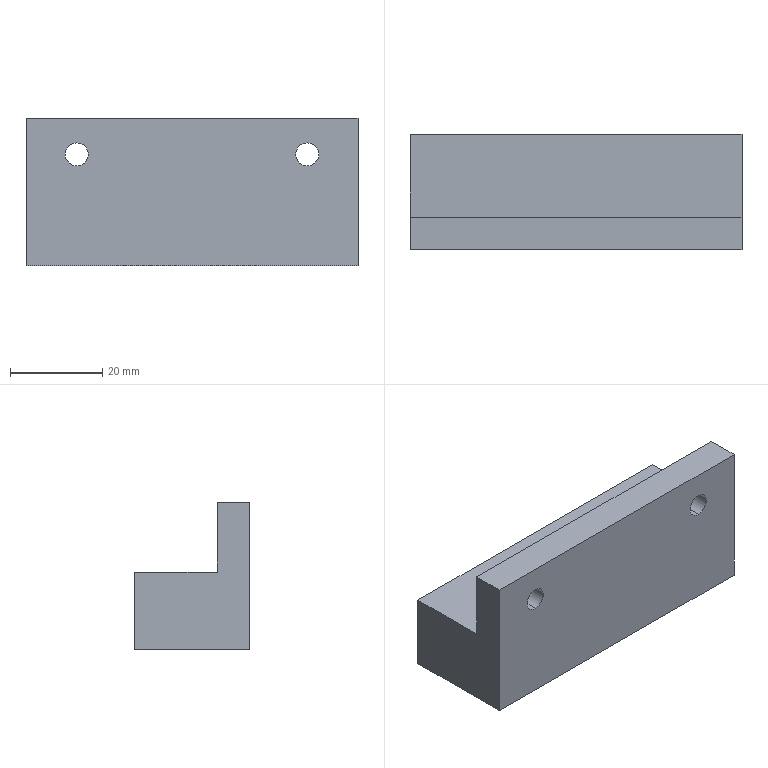Component | SolidWorks | LegSupport2-1 | 1 solid | 20 faces | box 72 x 25 x 32 mm | volume 37108 mm3 | cylinder 8 | plane 8 | cone 4 | commonest cylinder face diameters 5 x8
build123d program:
from build123d import *

# Parameters (mm, degrees)
SKETCH1_W             = 72
SKETCH1_H             = 32
BOSS_EXTRUDE1_DEPTH   = 25
SKETCH2_W             = 72
SKETCH2_H             = 15.16
CUT_EXTRUDE1_DEPTH    = 18
M5_TAPPED_HOLE1_D     = 5
M5_TAPPED_HOLE1_DEPTH = 14
M5_TAPPED_HOLE1_TIP   = 1.502
SKETCH7_R             = 2.5
CUT_EXTRUDE2_DEPTH    = 44.313


with BuildPart() as part:
    # Sketch1 → Boss-Extrude1 (new body)
    with BuildSketch(Plane(origin=(0, 0, 0), x_dir=(1, 0, 0), z_dir=(0, 1, 0))):
        Rectangle(SKETCH1_W, SKETCH1_H)
    extrude(amount=BOSS_EXTRUDE1_DEPTH)

    # Sketch2 → Cut-Extrude1 (cut)
    with BuildSketch(Plane(origin=(0, 25, 0), x_dir=(1, 0, 0), z_dir=(0, 1, 0))):
        with Locations((0, 8.42)):
            Rectangle(SKETCH2_W, SKETCH2_H)
    extrude(amount=-CUT_EXTRUDE1_DEPTH, mode=Mode.SUBTRACT)

    # M5 Tapped Hole1
    with Locations(Plane(origin=(-25, 25, 8.16), x_dir=(0, 0, 1), z_dir=(0, 1, 0))):
        with Locations((0, 0), (0, 50)):
            Hole(M5_TAPPED_HOLE1_D / 2, depth=M5_TAPPED_HOLE1_DEPTH)
            with Locations((0, 0, -(M5_TAPPED_HOLE1_DEPTH + M5_TAPPED_HOLE1_TIP / 2))):  # 118° drill point
                Cone(0, M5_TAPPED_HOLE1_D / 2, M5_TAPPED_HOLE1_TIP, mode=Mode.SUBTRACT)

    # Sketch7 → Cut-Extrude2 (cut, through all)
    with BuildSketch(Plane(origin=(0, 7, 0), x_dir=(1, 0, 0), z_dir=(0, 1, 0))):
        with Locations(Location((-25, 8.16, 0), (0, 0, 270))):
            Circle(SKETCH7_R)
        with Locations(Location((25, 8.16, 0), (0, 0, 90))):
            Circle(SKETCH7_R)
    extrude(amount=-CUT_EXTRUDE2_DEPTH, mode=Mode.SUBTRACT)


solid = part.part

# Placed as in the assembly
solid = solid.moved(Location((-96.534, 53.266, -102.347), (-180, 0, 180)))
STEP:
#1=COLOUR_RGB('',0.7922,0.8196,0.9333);
#2=FILL_AREA_STYLE_COLOUR('',#1);
#3=FILL_AREA_STYLE('',(#2));
#4=SURFACE_STYLE_FILL_AREA(#3);
#5=SURFACE_SIDE_STYLE('',(#4));
#6=SURFACE_STYLE_USAGE(.BOTH.,#5);
#7=PRESENTATION_STYLE_ASSIGNMENT((#6));
#8=CARTESIAN_POINT('',(-4.785,2.097,-3.61));
#9=VERTEX_POINT('',#8);
#10=CARTESIAN_POINT('',(-4.785,2.097,-3.807));
#11=VERTEX_POINT('',#10);
#12=CARTESIAN_POINT('',(-4.785,2.097,-3.708));
#13=DIRECTION('',(0.,1.,0.));
#14=DIRECTION('',(0.,0.,1.));
#15=AXIS2_PLACEMENT_3D('',#12,#13,#14);
#16=CIRCLE('',#15,0.09843);
#17=EDGE_CURVE('',#9,#11,#16,.T.);
#18=ORIENTED_EDGE('',*,*,#17,.F.);
#19=CARTESIAN_POINT('',(-4.785,2.373,-3.61));
#20=VERTEX_POINT('',#19);
#21=CARTESIAN_POINT('',(-4.785,2.097,-3.61));
#22=DIRECTION('',(0.,1.,0.));
#23=VECTOR('',#22,39.37);
#24=LINE('',#21,#23);
#25=EDGE_CURVE('',#9,#20,#24,.T.);
#26=ORIENTED_EDGE('',*,*,#25,.T.);
#27=CARTESIAN_POINT('',(-4.785,2.373,-3.807));
#28=VERTEX_POINT('',#27);
#29=CARTESIAN_POINT('',(-4.785,2.373,-3.708));
#30=DIRECTION('',(0.,1.,0.));
#31=DIRECTION('',(0.,0.,1.));
#32=AXIS2_PLACEMENT_3D('',#29,#30,#31);
#33=CIRCLE('',#32,0.09843);
#34=EDGE_CURVE('',#20,#28,#33,.T.);
#35=ORIENTED_EDGE('',*,*,#34,.T.);
#36=CARTESIAN_POINT('',(-4.785,2.097,-3.807));
#37=DIRECTION('',(0.,1.,0.));
#38=VECTOR('',#37,39.37);
#39=LINE('',#36,#38);
#40=EDGE_CURVE('',#11,#28,#39,.T.);
#41=ORIENTED_EDGE('',*,*,#40,.F.);
#42=EDGE_LOOP('',(#18,#26,#35,#41));
#43=FACE_OUTER_BOUND('',#42,.T.);
#44=CARTESIAN_POINT('',(-4.785,2.097,-3.708));
#45=DIRECTION('',(0.,1.,0.));
#46=DIRECTION('',(0.,0.,-1.));
#47=AXIS2_PLACEMENT_3D('',#44,#45,#46);
#48=CYLINDRICAL_SURFACE('',#47,0.09843);
#49=ADVANCED_FACE('',(#43),#48,.F.);
#50=CARTESIAN_POINT('',(-2.816,2.097,-3.61));
#51=VERTEX_POINT('',#50);
#52=CARTESIAN_POINT('',(-2.816,2.097,-3.807));
#53=VERTEX_POINT('',#52);
#54=CARTESIAN_POINT('',(-2.816,2.097,-3.708));
#55=DIRECTION('',(0.,1.,0.));
#56=DIRECTION('',(0.,0.,-1.));
#57=AXIS2_PLACEMENT_3D('',#54,#55,#56);
#58=CIRCLE('',#57,0.09843);
#59=EDGE_CURVE('',#51,#53,#58,.T.);
#60=ORIENTED_EDGE('',*,*,#59,.F.);
#61=CARTESIAN_POINT('',(-2.816,2.373,-3.61));
#62=VERTEX_POINT('',#61);
#63=CARTESIAN_POINT('',(-2.816,2.097,-3.61));
#64=DIRECTION('',(0.,1.,0.));
#65=VECTOR('',#64,39.37);
#66=LINE('',#63,#65);
#67=EDGE_CURVE('',#51,#62,#66,.T.);
#68=ORIENTED_EDGE('',*,*,#67,.T.);
#69=CARTESIAN_POINT('',(-2.816,2.373,-3.807));
#70=VERTEX_POINT('',#69);
#71=CARTESIAN_POINT('',(-2.816,2.373,-3.708));
#72=DIRECTION('',(0.,1.,0.));
#73=DIRECTION('',(0.,0.,-1.));
#74=AXIS2_PLACEMENT_3D('',#71,#72,#73);
#75=CIRCLE('',#74,0.09843);
#76=EDGE_CURVE('',#62,#70,#75,.T.);
#77=ORIENTED_EDGE('',*,*,#76,.T.);
#78=CARTESIAN_POINT('',(-2.816,2.097,-3.807));
#79=DIRECTION('',(0.,1.,0.));
#80=VECTOR('',#79,39.37);
#81=LINE('',#78,#80);
#82=EDGE_CURVE('',#53,#70,#81,.T.);
#83=ORIENTED_EDGE('',*,*,#82,.F.);
#84=EDGE_LOOP('',(#60,#68,#77,#83));
#85=FACE_OUTER_BOUND('',#84,.T.);
#86=CARTESIAN_POINT('',(-2.816,2.097,-3.708));
#87=DIRECTION('',(0.,1.,0.));
#88=DIRECTION('',(0.,0.,-1.));
#89=AXIS2_PLACEMENT_3D('',#86,#87,#88);
#90=CYLINDRICAL_SURFACE('',#89,0.09843);
#91=ADVANCED_FACE('',(#85),#90,.F.);
#92=CARTESIAN_POINT('',(-2.816,2.53,-4.252));
#93=VERTEX_POINT('',#92);
#94=CARTESIAN_POINT('',(-2.816,2.53,-4.449));
#95=VERTEX_POINT('',#94);
#96=CARTESIAN_POINT('',(-2.816,2.53,-4.351));
#97=DIRECTION('',(0.,1.,0.));
#98=DIRECTION('',(0.,0.,-1.));
#99=AXIS2_PLACEMENT_3D('',#96,#97,#98);
#100=CIRCLE('',#99,0.09843);
#101=EDGE_CURVE('',#93,#95,#100,.T.);
#102=ORIENTED_EDGE('',*,*,#101,.F.);
#103=CARTESIAN_POINT('',(-2.816,3.081,-4.252));
#104=VERTEX_POINT('',#103);
#105=CARTESIAN_POINT('',(-2.816,3.081,-4.252));
#106=DIRECTION('',(0.,1.,0.));
#107=VECTOR('',#106,39.37);
#108=LINE('',#105,#107);
#109=EDGE_CURVE('',#93,#104,#108,.T.);
#110=ORIENTED_EDGE('',*,*,#109,.T.);
#111=CARTESIAN_POINT('',(-2.816,3.081,-4.449));
#112=VERTEX_POINT('',#111);
#113=CARTESIAN_POINT('',(-2.816,3.081,-4.351));
#114=DIRECTION('',(0.,1.,0.));
#115=DIRECTION('',(0.,0.,-1.));
#116=AXIS2_PLACEMENT_3D('',#113,#114,#115);
#117=CIRCLE('',#116,0.09843);
#118=EDGE_CURVE('',#104,#112,#117,.T.);
#119=ORIENTED_EDGE('',*,*,#118,.T.);
#120=CARTESIAN_POINT('',(-2.816,3.081,-4.449));
#121=DIRECTION('',(0.,1.,0.));
#122=VECTOR('',#121,39.37);
#123=LINE('',#120,#122);
#124=EDGE_CURVE('',#95,#112,#123,.T.);
#125=ORIENTED_EDGE('',*,*,#124,.F.);
#126=EDGE_LOOP('',(#102,#110,#119,#125));
#127=FACE_OUTER_BOUND('',#126,.T.);
#128=CARTESIAN_POINT('',(-2.816,3.081,-4.351));
#129=DIRECTION('',(0.,1.,0.));
#130=DIRECTION('',(0.,0.,-1.));
#131=AXIS2_PLACEMENT_3D('',#128,#129,#130);
#132=CYLINDRICAL_SURFACE('',#131,0.09843);
#133=ADVANCED_FACE('',(#127),#132,.F.);
#134=CARTESIAN_POINT('',(-2.816,2.471,-4.351));
#135=VERTEX_POINT('',#134);
#136=CARTESIAN_POINT('',(-2.816,2.53,-4.449));
#137=DIRECTION('',(-0.,0.515,-0.8572));
#138=VECTOR('',#137,39.37);
#139=LINE('',#136,#138);
#140=EDGE_CURVE('',#135,#95,#139,.T.);
#141=ORIENTED_EDGE('',*,*,#140,.F.);
#142=CARTESIAN_POINT('',(-2.816,2.53,-4.252));
#143=DIRECTION('',(0.,0.515,0.8572));
#144=VECTOR('',#143,39.37);
#145=LINE('',#142,#144);
#146=EDGE_CURVE('',#135,#93,#145,.T.);
#147=ORIENTED_EDGE('',*,*,#146,.T.);
#148=ORIENTED_EDGE('',*,*,#101,.T.);
#149=EDGE_LOOP('',(#141,#147,#148));
#150=FACE_OUTER_BOUND('',#149,.T.);
#151=CARTESIAN_POINT('',(-2.816,2.53,-4.351));
#152=DIRECTION('',(0.,1.,0.));
#153=DIRECTION('',(0.,0.,-1.));
#154=AXIS2_PLACEMENT_3D('',#151,#152,#153);
#155=CONICAL_SURFACE('',#154,0.09843,1.03);
#156=ADVANCED_FACE('',(#150),#155,.F.);
#157=CARTESIAN_POINT('',(-4.785,2.53,-4.252));
#158=VERTEX_POINT('',#157);
#159=CARTESIAN_POINT('',(-4.785,2.53,-4.449));
#160=VERTEX_POINT('',#159);
#161=CARTESIAN_POINT('',(-4.785,2.53,-4.351));
#162=DIRECTION('',(0.,1.,0.));
#163=DIRECTION('',(0.,0.,-1.));
#164=AXIS2_PLACEMENT_3D('',#161,#162,#163);
#165=CIRCLE('',#164,0.09843);
#166=EDGE_CURVE('',#158,#160,#165,.T.);
#167=ORIENTED_EDGE('',*,*,#166,.F.);
#168=CARTESIAN_POINT('',(-4.785,3.081,-4.252));
#169=VERTEX_POINT('',#168);
#170=CARTESIAN_POINT('',(-4.785,3.081,-4.252));
#171=DIRECTION('',(0.,1.,0.));
#172=VECTOR('',#171,39.37);
#173=LINE('',#170,#172);
#174=EDGE_CURVE('',#158,#169,#173,.T.);
#175=ORIENTED_EDGE('',*,*,#174,.T.);
#176=CARTESIAN_POINT('',(-4.785,3.081,-4.449));
#177=VERTEX_POINT('',#176);
#178=CARTESIAN_POINT('',(-4.785,3.081,-4.351));
#179=DIRECTION('',(0.,1.,0.));
#180=DIRECTION('',(0.,0.,-1.));
#181=AXIS2_PLACEMENT_3D('',#178,#179,#180);
#182=CIRCLE('',#181,0.09843);
#183=EDGE_CURVE('',#169,#177,#182,.T.);
#184=ORIENTED_EDGE('',*,*,#183,.T.);
#185=CARTESIAN_POINT('',(-4.785,3.081,-4.449));
#186=DIRECTION('',(0.,1.,0.));
#187=VECTOR('',#186,39.37);
#188=LINE('',#185,#187);
#189=EDGE_CURVE('',#160,#177,#188,.T.);
#190=ORIENTED_EDGE('',*,*,#189,.F.);
#191=EDGE_LOOP('',(#167,#175,#184,#190));
#192=FACE_OUTER_BOUND('',#191,.T.);
#193=CARTESIAN_POINT('',(-4.785,3.081,-4.351));
#194=DIRECTION('',(0.,1.,0.));
#195=DIRECTION('',(0.,0.,-1.));
#196=AXIS2_PLACEMENT_3D('',#193,#194,#195);
#197=CYLINDRICAL_SURFACE('',#196,0.09843);
#198=ADVANCED_FACE('',(#192),#197,.F.);
#199=CARTESIAN_POINT('',(-4.785,2.471,-4.351));
#200=VERTEX_POINT('',#199);
#201=CARTESIAN_POINT('',(-4.785,2.53,-4.449));
#202=DIRECTION('',(-0.,0.515,-0.8572));
#203=VECTOR('',#202,39.37);
#204=LINE('',#201,#203);
#205=EDGE_CURVE('',#200,#160,#204,.T.);
#206=ORIENTED_EDGE('',*,*,#205,.F.);
#207=CARTESIAN_POINT('',(-4.785,2.53,-4.252));
#208=DIRECTION('',(0.,0.515,0.8572));
#209=VECTOR('',#208,39.37);
#210=LINE('',#207,#209);
#211=EDGE_CURVE('',#200,#158,#210,.T.);
#212=ORIENTED_EDGE('',*,*,#211,.T.);
#213=ORIENTED_EDGE('',*,*,#166,.T.);
#214=EDGE_LOOP('',(#206,#212,#213));
#215=FACE_OUTER_BOUND('',#214,.T.);
#216=CARTESIAN_POINT('',(-4.785,2.53,-4.351));
#217=DIRECTION('',(0.,1.,0.));
#218=DIRECTION('',(0.,0.,-1.));
#219=AXIS2_PLACEMENT_3D('',#216,#217,#218);
#220=CONICAL_SURFACE('',#219,0.09843,1.03);
#221=ADVANCED_FACE('',(#215),#220,.F.);
#222=CARTESIAN_POINT('',(-5.218,2.373,-3.399));
#223=VERTEX_POINT('',#222);
#224=CARTESIAN_POINT('',(-2.383,2.373,-3.399));
#225=VERTEX_POINT('',#224);
#226=CARTESIAN_POINT('',(-2.383,2.373,-3.399));
#227=DIRECTION('',(1.,0.,-0.));
#228=VECTOR('',#227,39.37);
#229=LINE('',#226,#228);
#230=EDGE_CURVE('',#223,#225,#229,.T.);
#231=ORIENTED_EDGE('',*,*,#230,.F.);
#232=CARTESIAN_POINT('',(-5.218,2.097,-3.399));
#233=VERTEX_POINT('',#232);
#234=CARTESIAN_POINT('',(-5.218,3.081,-3.399));
#235=DIRECTION('',(0.,-1.,0.));
#236=VECTOR('',#235,39.37);
#237=LINE('',#234,#236);
#238=EDGE_CURVE('',#223,#233,#237,.T.);
#239=ORIENTED_EDGE('',*,*,#238,.T.);
#240=CARTESIAN_POINT('',(-2.383,2.097,-3.399));
#241=VERTEX_POINT('',#240);
#242=CARTESIAN_POINT('',(-2.383,2.097,-3.399));
#243=DIRECTION('',(1.,0.,-0.));
#244=VECTOR('',#243,39.37);
#245=LINE('',#242,#244);
#246=EDGE_CURVE('',#233,#241,#245,.T.);
#247=ORIENTED_EDGE('',*,*,#246,.T.);
#248=CARTESIAN_POINT('',(-2.383,3.081,-3.399));
#249=DIRECTION('',(0.,-1.,0.));
#250=VECTOR('',#249,39.37);
#251=LINE('',#248,#250);
#252=EDGE_CURVE('',#225,#241,#251,.T.);
#253=ORIENTED_EDGE('',*,*,#252,.F.);
#254=EDGE_LOOP('',(#231,#239,#247,#253));
#255=FACE_OUTER_BOUND('',#254,.T.);
#256=CARTESIAN_POINT('',(-2.383,3.081,-3.399));
#257=DIRECTION('',(-0.,0.,-1.));
#258=DIRECTION('',(-1.,0.,0.));
#259=AXIS2_PLACEMENT_3D('',#256,#257,#258);
#260=PLANE('',#259);
#261=ADVANCED_FACE('',(#255),#260,.F.);
#262=CARTESIAN_POINT('',(-5.218,2.373,-3.996));
#263=VERTEX_POINT('',#262);
#264=CARTESIAN_POINT('',(-5.218,2.373,-3.399));
#265=DIRECTION('',(0.,0.,1.));
#266=VECTOR('',#265,39.37);
#267=LINE('',#264,#266);
#268=EDGE_CURVE('',#263,#223,#267,.T.);
#269=ORIENTED_EDGE('',*,*,#268,.F.);
#270=CARTESIAN_POINT('',(-5.218,3.081,-3.996));
#271=VERTEX_POINT('',#270);
#272=CARTESIAN_POINT('',(-5.218,2.373,-3.996));
#273=DIRECTION('',(0.,1.,0.));
#274=VECTOR('',#273,39.37);
#275=LINE('',#272,#274);
#276=EDGE_CURVE('',#263,#271,#275,.T.);
#277=ORIENTED_EDGE('',*,*,#276,.T.);
#278=CARTESIAN_POINT('',(-5.218,3.081,-4.659));
#279=VERTEX_POINT('',#278);
#280=CARTESIAN_POINT('',(-5.218,3.081,-3.399));
#281=DIRECTION('',(0.,0.,1.));
#282=VECTOR('',#281,39.37);
#283=LINE('',#280,#282);
#284=EDGE_CURVE('',#279,#271,#283,.T.);
#285=ORIENTED_EDGE('',*,*,#284,.F.);
#286=CARTESIAN_POINT('',(-5.218,2.097,-4.659));
#287=VERTEX_POINT('',#286);
#288=CARTESIAN_POINT('',(-5.218,3.081,-4.659));
#289=DIRECTION('',(0.,-1.,0.));
#290=VECTOR('',#289,39.37);
#291=LINE('',#288,#290);
#292=EDGE_CURVE('',#279,#287,#291,.T.);
#293=ORIENTED_EDGE('',*,*,#292,.T.);
#294=CARTESIAN_POINT('',(-5.218,2.097,-3.399));
#295=DIRECTION('',(0.,0.,1.));
#296=VECTOR('',#295,39.37);
#297=LINE('',#294,#296);
#298=EDGE_CURVE('',#287,#233,#297,.T.);
#299=ORIENTED_EDGE('',*,*,#298,.T.);
#300=ORIENTED_EDGE('',*,*,#238,.F.);
#301=EDGE_LOOP('',(#269,#277,#285,#293,#299,#300));
#302=FACE_OUTER_BOUND('',#301,.T.);
#303=CARTESIAN_POINT('',(-5.218,3.081,-3.399));
#304=DIRECTION('',(1.,0.,-0.));
#305=DIRECTION('',(-0.,0.,-1.));
#306=AXIS2_PLACEMENT_3D('',#303,#304,#305);
#307=PLANE('',#306);
#308=ADVANCED_FACE('',(#302),#307,.F.);
#309=CARTESIAN_POINT('',(-2.383,3.081,-3.996));
#310=VERTEX_POINT('',#309);
#311=CARTESIAN_POINT('',(-2.383,3.081,-4.659));
#312=VERTEX_POINT('',#311);
#313=CARTESIAN_POINT('',(-2.383,3.081,-3.399));
#314=DIRECTION('',(-0.,0.,-1.));
#315=VECTOR('',#314,39.37);
#316=LINE('',#313,#315);
#317=EDGE_CURVE('',#310,#312,#316,.T.);
#318=ORIENTED_EDGE('',*,*,#317,.F.);
#319=CARTESIAN_POINT('',(-2.383,2.373,-3.996));
#320=VERTEX_POINT('',#319);
#321=CARTESIAN_POINT('',(-2.383,2.373,-3.996));
#322=DIRECTION('',(0.,1.,0.));
#323=VECTOR('',#322,39.37);
#324=LINE('',#321,#323);
#325=EDGE_CURVE('',#320,#310,#324,.T.);
#326=ORIENTED_EDGE('',*,*,#325,.F.);
#327=CARTESIAN_POINT('',(-2.383,2.373,-3.399));
#328=DIRECTION('',(-0.,0.,-1.));
#329=VECTOR('',#328,39.37);
#330=LINE('',#327,#329);
#331=EDGE_CURVE('',#225,#320,#330,.T.);
#332=ORIENTED_EDGE('',*,*,#331,.F.);
#333=ORIENTED_EDGE('',*,*,#252,.T.);
#334=CARTESIAN_POINT('',(-2.383,2.097,-4.659));
#335=VERTEX_POINT('',#334);
#336=CARTESIAN_POINT('',(-2.383,2.097,-3.399));
#337=DIRECTION('',(-0.,0.,-1.));
#338=VECTOR('',#337,39.37);
#339=LINE('',#336,#338);
#340=EDGE_CURVE('',#241,#335,#339,.T.);
#341=ORIENTED_EDGE('',*,*,#340,.T.);
#342=CARTESIAN_POINT('',(-2.383,3.081,-4.659));
#343=DIRECTION('',(0.,-1.,0.));
#344=VECTOR('',#343,39.37);
#345=LINE('',#342,#344);
#346=EDGE_CURVE('',#312,#335,#345,.T.);
#347=ORIENTED_EDGE('',*,*,#346,.F.);
#348=EDGE_LOOP('',(#318,#326,#332,#333,#341,#347));
#349=FACE_OUTER_BOUND('',#348,.T.);
#350=CARTESIAN_POINT('',(-2.383,3.081,-3.399));
#351=DIRECTION('',(-1.,0.,0.));
#352=DIRECTION('',(0.,0.,1.));
#353=AXIS2_PLACEMENT_3D('',#350,#351,#352);
#354=PLANE('',#353);
#355=ADVANCED_FACE('',(#349),#354,.F.);
#356=CARTESIAN_POINT('',(-2.383,2.097,-4.659));
#357=DIRECTION('',(-1.,0.,0.));
#358=VECTOR('',#357,39.37);
#359=LINE('',#356,#358);
#360=EDGE_CURVE('',#335,#287,#359,.T.);
#361=ORIENTED_EDGE('',*,*,#360,.T.);
#362=ORIENTED_EDGE('',*,*,#292,.F.);
#363=CARTESIAN_POINT('',(-2.383,3.081,-4.659));
#364=DIRECTION('',(-1.,0.,0.));
#365=VECTOR('',#364,39.37);
#366=LINE('',#363,#365);
#367=EDGE_CURVE('',#312,#279,#366,.T.);
#368=ORIENTED_EDGE('',*,*,#367,.F.);
#369=ORIENTED_EDGE('',*,*,#346,.T.);
#370=EDGE_LOOP('',(#361,#362,#368,#369));
#371=FACE_OUTER_BOUND('',#370,.T.);
#372=CARTESIAN_POINT('',(-2.383,3.081,-4.659));
#373=DIRECTION('',(0.,0.,1.));
#374=DIRECTION('',(1.,0.,-0.));
#375=AXIS2_PLACEMENT_3D('',#372,#373,#374);
#376=PLANE('',#375);
#377=ADVANCED_FACE('',(#371),#376,.F.);
#378=CARTESIAN_POINT('',(-2.816,3.081,-4.351));
#379=DIRECTION('',(0.,1.,0.));
#380=DIRECTION('',(0.,0.,-1.));
#381=AXIS2_PLACEMENT_3D('',#378,#379,#380);
#382=CIRCLE('',#381,0.09843);
#383=EDGE_CURVE('',#112,#104,#382,.T.);
#384=ORIENTED_EDGE('',*,*,#383,.F.);
#385=ORIENTED_EDGE('',*,*,#118,.F.);
#386=EDGE_LOOP('',(#384,#385));
#387=FACE_BOUND('',#386,.T.);
#388=CARTESIAN_POINT('',(-4.785,3.081,-4.351));
#389=DIRECTION('',(0.,1.,0.));
#390=DIRECTION('',(0.,0.,-1.));
#391=AXIS2_PLACEMENT_3D('',#388,#389,#390);
#392=CIRCLE('',#391,0.09843);
#393=EDGE_CURVE('',#177,#169,#392,.T.);
#394=ORIENTED_EDGE('',*,*,#393,.F.);
#395=ORIENTED_EDGE('',*,*,#183,.F.);
#396=EDGE_LOOP('',(#394,#395));
#397=FACE_BOUND('',#396,.T.);
#398=CARTESIAN_POINT('',(-2.383,3.081,-3.996));
#399=DIRECTION('',(-1.,0.,0.));
#400=VECTOR('',#399,39.37);
#401=LINE('',#398,#400);
#402=EDGE_CURVE('',#310,#271,#401,.T.);
#403=ORIENTED_EDGE('',*,*,#402,.F.);
#404=ORIENTED_EDGE('',*,*,#317,.T.);
#405=ORIENTED_EDGE('',*,*,#367,.T.);
#406=ORIENTED_EDGE('',*,*,#284,.T.);
#407=EDGE_LOOP('',(#403,#404,#405,#406));
#408=FACE_OUTER_BOUND('',#407,.T.);
#409=CARTESIAN_POINT('',(-3.801,3.081,-4.029));
#410=DIRECTION('',(0.,1.,0.));
#411=DIRECTION('',(-0.,0.,-1.));
#412=AXIS2_PLACEMENT_3D('',#409,#410,#411);
#413=PLANE('',#412);
#414=ADVANCED_FACE('',(#387,#397,#408),#413,.T.);
#415=CARTESIAN_POINT('',(-4.785,2.097,-3.708));
#416=DIRECTION('',(0.,1.,0.));
#417=DIRECTION('',(0.,0.,1.));
#418=AXIS2_PLACEMENT_3D('',#415,#416,#417);
#419=CIRCLE('',#418,0.09843);
#420=EDGE_CURVE('',#11,#9,#419,.T.);
#421=ORIENTED_EDGE('',*,*,#420,.T.);
#422=ORIENTED_EDGE('',*,*,#17,.T.);
#423=EDGE_LOOP('',(#421,#422));
#424=FACE_BOUND('',#423,.T.);
#425=CARTESIAN_POINT('',(-2.816,2.097,-3.708));
#426=DIRECTION('',(0.,1.,0.));
#427=DIRECTION('',(0.,0.,-1.));
#428=AXIS2_PLACEMENT_3D('',#425,#426,#427);
#429=CIRCLE('',#428,0.09843);
#430=EDGE_CURVE('',#53,#51,#429,.T.);
#431=ORIENTED_EDGE('',*,*,#430,.T.);
#432=ORIENTED_EDGE('',*,*,#59,.T.);
#433=EDGE_LOOP('',(#431,#432));
#434=FACE_BOUND('',#433,.T.);
#435=ORIENTED_EDGE('',*,*,#298,.F.);
#436=ORIENTED_EDGE('',*,*,#360,.F.);
#437=ORIENTED_EDGE('',*,*,#340,.F.);
#438=ORIENTED_EDGE('',*,*,#246,.F.);
#439=EDGE_LOOP('',(#435,#436,#437,#438));
#440=FACE_OUTER_BOUND('',#439,.T.);
#441=CARTESIAN_POINT('',(-3.801,2.097,-4.029));
#442=DIRECTION('',(0.,1.,0.));
#443=DIRECTION('',(-0.,0.,-1.));
#444=AXIS2_PLACEMENT_3D('',#441,#442,#443);
#445=PLANE('',#444);
#446=ADVANCED_FACE('',(#424,#434,#440),#445,.F.);
#447=ORIENTED_EDGE('',*,*,#402,.T.);
#448=ORIENTED_EDGE('',*,*,#276,.F.);
#449=CARTESIAN_POINT('',(-2.383,2.373,-3.996));
#450=DIRECTION('',(-1.,0.,0.));
#451=VECTOR('',#450,39.37);
#452=LINE('',#449,#451);
#453=EDGE_CURVE('',#320,#263,#452,.T.);
#454=ORIENTED_EDGE('',*,*,#453,.F.);
#455=ORIENTED_EDGE('',*,*,#325,.T.);
#456=EDGE_LOOP('',(#447,#448,#454,#455));
#457=FACE_OUTER_BOUND('',#456,.T.);
#458=CARTESIAN_POINT('',(-2.383,2.373,-3.996));
#459=DIRECTION('',(-0.,0.,-1.));
#460=DIRECTION('',(-1.,0.,0.));
#461=AXIS2_PLACEMENT_3D('',#458,#459,#460);
#462=PLANE('',#461);
#463=ADVANCED_FACE('',(#457),#462,.F.);
#464=CARTESIAN_POINT('',(-4.785,2.373,-3.708));
#465=DIRECTION('',(0.,1.,0.));
#466=DIRECTION('',(0.,0.,1.));
#467=AXIS2_PLACEMENT_3D('',#464,#465,#466);
#468=CIRCLE('',#467,0.09843);
#469=EDGE_CURVE('',#28,#20,#468,.T.);
#470=ORIENTED_EDGE('',*,*,#469,.F.);
#471=ORIENTED_EDGE('',*,*,#34,.F.);
#472=EDGE_LOOP('',(#470,#471));
#473=FACE_BOUND('',#472,.T.);
#474=CARTESIAN_POINT('',(-2.816,2.373,-3.708));
#475=DIRECTION('',(0.,1.,0.));
#476=DIRECTION('',(0.,0.,-1.));
#477=AXIS2_PLACEMENT_3D('',#474,#475,#476);
#478=CIRCLE('',#477,0.09843);
#479=EDGE_CURVE('',#70,#62,#478,.T.);
#480=ORIENTED_EDGE('',*,*,#479,.F.);
#481=ORIENTED_EDGE('',*,*,#76,.F.);
#482=EDGE_LOOP('',(#480,#481));
#483=FACE_BOUND('',#482,.T.);
#484=ORIENTED_EDGE('',*,*,#331,.T.);
#485=ORIENTED_EDGE('',*,*,#453,.T.);
#486=ORIENTED_EDGE('',*,*,#268,.T.);
#487=ORIENTED_EDGE('',*,*,#230,.T.);
#488=EDGE_LOOP('',(#484,#485,#486,#487));
#489=FACE_OUTER_BOUND('',#488,.T.);
#490=CARTESIAN_POINT('',(-3.801,2.373,-4.029));
#491=DIRECTION('',(0.,1.,0.));
#492=DIRECTION('',(-0.,0.,-1.));
#493=AXIS2_PLACEMENT_3D('',#490,#491,#492);
#494=PLANE('',#493);
#495=ADVANCED_FACE('',(#473,#483,#489),#494,.T.);
#496=ORIENTED_EDGE('',*,*,#211,.F.);
#497=ORIENTED_EDGE('',*,*,#205,.T.);
#498=CARTESIAN_POINT('',(-4.785,2.53,-4.351));
#499=DIRECTION('',(0.,1.,0.));
#500=DIRECTION('',(0.,0.,-1.));
#501=AXIS2_PLACEMENT_3D('',#498,#499,#500);
#502=CIRCLE('',#501,0.09843);
#503=EDGE_CURVE('',#160,#158,#502,.T.);
#504=ORIENTED_EDGE('',*,*,#503,.T.);
#505=EDGE_LOOP('',(#496,#497,#504));
#506=FACE_OUTER_BOUND('',#505,.T.);
#507=CARTESIAN_POINT('',(-4.785,2.53,-4.351));
#508=DIRECTION('',(0.,1.,0.));
#509=DIRECTION('',(0.,0.,-1.));
#510=AXIS2_PLACEMENT_3D('',#507,#508,#509);
#511=CONICAL_SURFACE('',#510,0.09843,1.03);
#512=ADVANCED_FACE('',(#506),#511,.F.);
#513=ORIENTED_EDGE('',*,*,#174,.F.);
#514=ORIENTED_EDGE('',*,*,#503,.F.);
#515=ORIENTED_EDGE('',*,*,#189,.T.);
#516=ORIENTED_EDGE('',*,*,#393,.T.);
#517=EDGE_LOOP('',(#513,#514,#515,#516));
#518=FACE_OUTER_BOUND('',#517,.T.);
#519=CARTESIAN_POINT('',(-4.785,3.081,-4.351));
#520=DIRECTION('',(0.,1.,0.));
#521=DIRECTION('',(0.,0.,-1.));
#522=AXIS2_PLACEMENT_3D('',#519,#520,#521);
#523=CYLINDRICAL_SURFACE('',#522,0.09843);
#524=ADVANCED_FACE('',(#518),#523,.F.);
#525=ORIENTED_EDGE('',*,*,#146,.F.);
#526=ORIENTED_EDGE('',*,*,#140,.T.);
#527=CARTESIAN_POINT('',(-2.816,2.53,-4.351));
#528=DIRECTION('',(0.,1.,0.));
#529=DIRECTION('',(0.,0.,-1.));
#530=AXIS2_PLACEMENT_3D('',#527,#528,#529);
#531=CIRCLE('',#530,0.09843);
#532=EDGE_CURVE('',#95,#93,#531,.T.);
#533=ORIENTED_EDGE('',*,*,#532,.T.);
#534=EDGE_LOOP('',(#525,#526,#533));
#535=FACE_OUTER_BOUND('',#534,.T.);
#536=CARTESIAN_POINT('',(-2.816,2.53,-4.351));
#537=DIRECTION('',(0.,1.,0.));
#538=DIRECTION('',(0.,0.,-1.));
#539=AXIS2_PLACEMENT_3D('',#536,#537,#538);
#540=CONICAL_SURFACE('',#539,0.09843,1.03);
#541=ADVANCED_FACE('',(#535),#540,.F.);
#542=ORIENTED_EDGE('',*,*,#109,.F.);
#543=ORIENTED_EDGE('',*,*,#532,.F.);
#544=ORIENTED_EDGE('',*,*,#124,.T.);
#545=ORIENTED_EDGE('',*,*,#383,.T.);
#546=EDGE_LOOP('',(#542,#543,#544,#545));
#547=FACE_OUTER_BOUND('',#546,.T.);
#548=CARTESIAN_POINT('',(-2.816,3.081,-4.351));
#549=DIRECTION('',(0.,1.,0.));
#550=DIRECTION('',(0.,0.,-1.));
#551=AXIS2_PLACEMENT_3D('',#548,#549,#550);
#552=CYLINDRICAL_SURFACE('',#551,0.09843);
#553=ADVANCED_FACE('',(#547),#552,.F.);
#554=ORIENTED_EDGE('',*,*,#67,.F.);
#555=ORIENTED_EDGE('',*,*,#430,.F.);
#556=ORIENTED_EDGE('',*,*,#82,.T.);
#557=ORIENTED_EDGE('',*,*,#479,.T.);
#558=EDGE_LOOP('',(#554,#555,#556,#557));
#559=FACE_OUTER_BOUND('',#558,.T.);
#560=CARTESIAN_POINT('',(-2.816,2.097,-3.708));
#561=DIRECTION('',(0.,1.,0.));
#562=DIRECTION('',(0.,0.,-1.));
#563=AXIS2_PLACEMENT_3D('',#560,#561,#562);
#564=CYLINDRICAL_SURFACE('',#563,0.09843);
#565=ADVANCED_FACE('',(#559),#564,.F.);
#566=ORIENTED_EDGE('',*,*,#25,.F.);
#567=ORIENTED_EDGE('',*,*,#420,.F.);
#568=ORIENTED_EDGE('',*,*,#40,.T.);
#569=ORIENTED_EDGE('',*,*,#469,.T.);
#570=EDGE_LOOP('',(#566,#567,#568,#569));
#571=FACE_OUTER_BOUND('',#570,.T.);
#572=CARTESIAN_POINT('',(-4.785,2.097,-3.708));
#573=DIRECTION('',(0.,1.,0.));
#574=DIRECTION('',(0.,0.,-1.));
#575=AXIS2_PLACEMENT_3D('',#572,#573,#574);
#576=CYLINDRICAL_SURFACE('',#575,0.09843);
#577=ADVANCED_FACE('',(#571),#576,.F.);
#578=CLOSED_SHELL('',(#49,#91,#133,#156,#198,#221,#261,#308,#355,#377,#414,#446,#463,#495,#512,#524,#541,#553,#565,#577));
#579=MANIFOLD_SOLID_BREP('',#578);
#580=STYLED_ITEM('',(#7),#579);
#581=PRESENTATION_LAYER_ASSIGNMENT('','',(#580));
#582=(LENGTH_UNIT()NAMED_UNIT(*)SI_UNIT($,.METRE.));
#583=LENGTH_MEASURE_WITH_UNIT(LENGTH_MEASURE(0.0254),#582);
#584=DIMENSIONAL_EXPONENTS(1.,0.,0.,0.,0.,0.,0.);
#585=(CONVERSION_BASED_UNIT('',#583)LENGTH_UNIT()NAMED_UNIT(#584));
#586=UNCERTAINTY_MEASURE_WITH_UNIT(LENGTH_MEASURE(0.00001),#585,'','');
#587=(NAMED_UNIT(*)PLANE_ANGLE_UNIT()SI_UNIT($,.RADIAN.));
#588=(NAMED_UNIT(*)SI_UNIT($,.STERADIAN.)SOLID_ANGLE_UNIT());
#589=(GEOMETRIC_REPRESENTATION_CONTEXT(3)GLOBAL_UNCERTAINTY_ASSIGNED_CONTEXT((#586))GLOBAL_UNIT_ASSIGNED_CONTEXT((#585,#587,#588))REPRESENTATION_CONTEXT('',''));
#590=MECHANICAL_DESIGN_GEOMETRIC_PRESENTATION_REPRESENTATION('',(#580),#589);
#591=CARTESIAN_POINT('',(0.,0.,0.));
#592=DIRECTION('',(0.,0.,1.));
#593=DIRECTION('',(1.,0.,0.));
#594=AXIS2_PLACEMENT_3D('',#591,#592,#593);
#595=(LENGTH_UNIT()NAMED_UNIT(*)SI_UNIT($,.METRE.));
#596=LENGTH_MEASURE_WITH_UNIT(LENGTH_MEASURE(0.0254),#595);
#597=DIMENSIONAL_EXPONENTS(1.,0.,0.,0.,0.,0.,0.);
#598=(CONVERSION_BASED_UNIT('',#596)LENGTH_UNIT()NAMED_UNIT(#597));
#599=UNCERTAINTY_MEASURE_WITH_UNIT(LENGTH_MEASURE(0.00001),#598,'','');
#600=(NAMED_UNIT(*)PLANE_ANGLE_UNIT()SI_UNIT($,.RADIAN.));
#601=(NAMED_UNIT(*)SI_UNIT($,.STERADIAN.)SOLID_ANGLE_UNIT());
#602=(GEOMETRIC_REPRESENTATION_CONTEXT(3)GLOBAL_UNCERTAINTY_ASSIGNED_CONTEXT((#599))GLOBAL_UNIT_ASSIGNED_CONTEXT((#598,#600,#601))REPRESENTATION_CONTEXT('',''));
#603=ADVANCED_BREP_SHAPE_REPRESENTATION('',(#579,#594),#602);